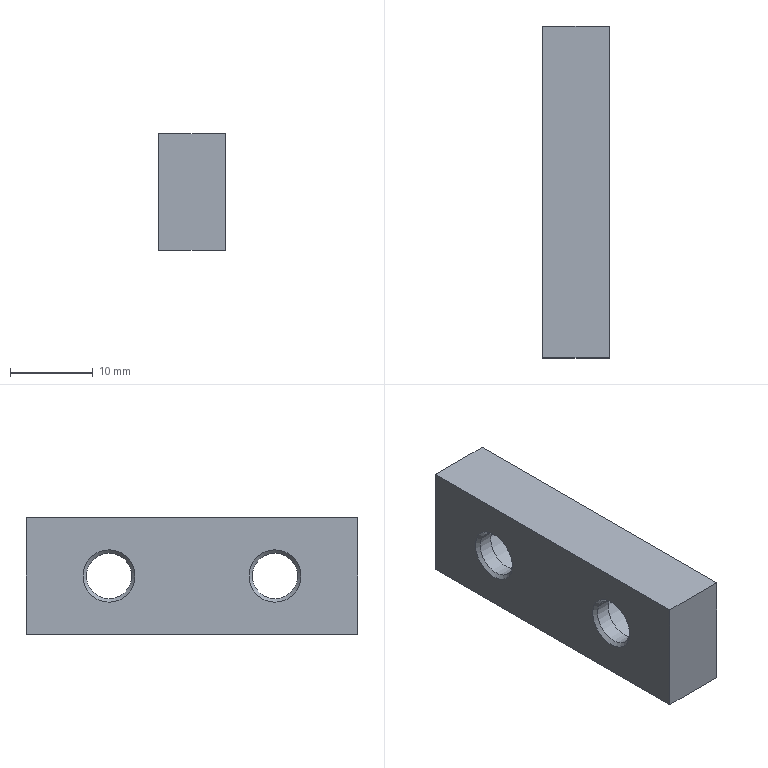Component | NX | A_SUPPORT_PLATE_2 | 1 solid | 16 faces | box 8 x 40 x 14 mm | volume 3456 mm3 | plane 8 | cylinder 4 | cone 4 | commonest cylinder face diameters 5.5 x2 10 x2
STEP:
#1=CARTESIAN_POINT('',(0.,0.,0.));
#2=DIRECTION('',(0.,0.,1.));
#3=DIRECTION('',(1.,0.,0.));
#4=AXIS2_PLACEMENT_3D('',#1,#2,#3);
#5=CARTESIAN_POINT('',(-25.,-20.,12.5));
#6=VERTEX_POINT('',#5);
#7=CARTESIAN_POINT('',(-25.,-20.,-1.5));
#8=VERTEX_POINT('',#7);
#9=CARTESIAN_POINT('',(-25.,-20.,12.5));
#10=DIRECTION('',(0.,0.,-1.));
#11=VECTOR('',#10,1.);
#12=LINE('',#9,#11);
#13=CARTESIAN_POINT('',(-33.,-20.,12.5));
#14=DIRECTION('',(0.,-1.,0.));
#15=DIRECTION('',(0.,0.,-1.));
#16=AXIS2_PLACEMENT_3D('',#13,#14,#15);
#17=PLANE('',#16);
#18=CARTESIAN_POINT('',(0.,8.));
#19=DIRECTION('',(1.,0.));
#20=VECTOR('',#19,1.);
#21=LINE('',#18,#20);
#22=(GEOMETRIC_REPRESENTATION_CONTEXT(2)PARAMETRIC_REPRESENTATION_CONTEXT()REPRESENTATION_CONTEXT('',''));
#23=DEFINITIONAL_REPRESENTATION('',(#21),#22);
#24=PCURVE('',#17,#23);
#25=CARTESIAN_POINT('',(-25.,0.,5.5));
#26=DIRECTION('',(1.,0.,0.));
#27=DIRECTION('',(0.,0.,-1.));
#28=AXIS2_PLACEMENT_3D('',#25,#26,#27);
#29=PLANE('',#28);
#30=CARTESIAN_POINT('',(-7.,-20.));
#31=DIRECTION('',(1.,0.));
#32=VECTOR('',#31,1.);
#33=LINE('',#30,#32);
#34=(GEOMETRIC_REPRESENTATION_CONTEXT(2)PARAMETRIC_REPRESENTATION_CONTEXT()REPRESENTATION_CONTEXT('',''));
#35=DEFINITIONAL_REPRESENTATION('',(#33),#34);
#36=PCURVE('',#29,#35);
#37=SURFACE_CURVE('',#12,(#24,#36),.PCURVE_S1.);
#38=EDGE_CURVE('',#6,#8,#37,.T.);
#39=ORIENTED_EDGE('',*,*,#38,.F.);
#40=CARTESIAN_POINT('',(-33.,-20.,12.5));
#41=VERTEX_POINT('',#40);
#42=CARTESIAN_POINT('',(-33.,-20.,12.5));
#43=DIRECTION('',(1.,0.,0.));
#44=VECTOR('',#43,1.);
#45=LINE('',#42,#44);
#46=CARTESIAN_POINT('',(0.,0.));
#47=DIRECTION('',(0.,1.));
#48=VECTOR('',#47,1.);
#49=LINE('',#46,#48);
#50=(GEOMETRIC_REPRESENTATION_CONTEXT(2)PARAMETRIC_REPRESENTATION_CONTEXT()REPRESENTATION_CONTEXT('',''));
#51=DEFINITIONAL_REPRESENTATION('',(#49),#50);
#52=PCURVE('',#17,#51);
#53=CARTESIAN_POINT('',(-33.,20.,12.5));
#54=DIRECTION('',(0.,0.,1.));
#55=DIRECTION('',(1.,0.,0.));
#56=AXIS2_PLACEMENT_3D('',#53,#54,#55);
#57=PLANE('',#56);
#58=CARTESIAN_POINT('',(0.,-40.));
#59=DIRECTION('',(1.,0.));
#60=VECTOR('',#59,1.);
#61=LINE('',#58,#60);
#62=(GEOMETRIC_REPRESENTATION_CONTEXT(2)PARAMETRIC_REPRESENTATION_CONTEXT()REPRESENTATION_CONTEXT('',''));
#63=DEFINITIONAL_REPRESENTATION('',(#61),#62);
#64=PCURVE('',#57,#63);
#65=SURFACE_CURVE('',#45,(#52,#64),.PCURVE_S1.);
#66=EDGE_CURVE('',#41,#6,#65,.T.);
#67=ORIENTED_EDGE('',*,*,#66,.F.);
#68=CARTESIAN_POINT('',(-33.,-20.,-1.5));
#69=VERTEX_POINT('',#68);
#70=CARTESIAN_POINT('',(-33.,-20.,12.5));
#71=DIRECTION('',(0.,0.,-1.));
#72=VECTOR('',#71,1.);
#73=LINE('',#70,#72);
#74=CARTESIAN_POINT('',(0.,0.));
#75=DIRECTION('',(1.,0.));
#76=VECTOR('',#75,1.);
#77=LINE('',#74,#76);
#78=(GEOMETRIC_REPRESENTATION_CONTEXT(2)PARAMETRIC_REPRESENTATION_CONTEXT()REPRESENTATION_CONTEXT('',''));
#79=DEFINITIONAL_REPRESENTATION('',(#77),#78);
#80=PCURVE('',#17,#79);
#81=CARTESIAN_POINT('',(-33.,0.,5.5));
#82=DIRECTION('',(1.,0.,0.));
#83=DIRECTION('',(0.,0.,-1.));
#84=AXIS2_PLACEMENT_3D('',#81,#82,#83);
#85=PLANE('',#84);
#86=CARTESIAN_POINT('',(-7.,-20.));
#87=DIRECTION('',(1.,0.));
#88=VECTOR('',#87,1.);
#89=LINE('',#86,#88);
#90=(GEOMETRIC_REPRESENTATION_CONTEXT(2)PARAMETRIC_REPRESENTATION_CONTEXT()REPRESENTATION_CONTEXT('',''));
#91=DEFINITIONAL_REPRESENTATION('',(#89),#90);
#92=PCURVE('',#85,#91);
#93=SURFACE_CURVE('',#73,(#80,#92),.PCURVE_S1.);
#94=EDGE_CURVE('',#41,#69,#93,.T.);
#95=ORIENTED_EDGE('',*,*,#94,.T.);
#96=CARTESIAN_POINT('',(-33.,-20.,-1.5));
#97=DIRECTION('',(1.,0.,0.));
#98=VECTOR('',#97,1.);
#99=LINE('',#96,#98);
#100=CARTESIAN_POINT('',(14.,0.));
#101=DIRECTION('',(0.,1.));
#102=VECTOR('',#101,1.);
#103=LINE('',#100,#102);
#104=(GEOMETRIC_REPRESENTATION_CONTEXT(2)PARAMETRIC_REPRESENTATION_CONTEXT()REPRESENTATION_CONTEXT('',''));
#105=DEFINITIONAL_REPRESENTATION('',(#103),#104);
#106=PCURVE('',#17,#105);
#107=CARTESIAN_POINT('',(-33.,-20.,-1.5));
#108=DIRECTION('',(0.,0.,-1.));
#109=DIRECTION('',(-1.,0.,0.));
#110=AXIS2_PLACEMENT_3D('',#107,#108,#109);
#111=PLANE('',#110);
#112=CARTESIAN_POINT('',(0.,0.));
#113=DIRECTION('',(-1.,0.));
#114=VECTOR('',#113,1.);
#115=LINE('',#112,#114);
#116=(GEOMETRIC_REPRESENTATION_CONTEXT(2)PARAMETRIC_REPRESENTATION_CONTEXT()REPRESENTATION_CONTEXT('',''));
#117=DEFINITIONAL_REPRESENTATION('',(#115),#116);
#118=PCURVE('',#111,#117);
#119=SURFACE_CURVE('',#99,(#106,#118),.PCURVE_S1.);
#120=EDGE_CURVE('',#69,#8,#119,.T.);
#121=ORIENTED_EDGE('',*,*,#120,.T.);
#122=EDGE_LOOP('',(#39,#67,#95,#121));
#123=FACE_BOUND('',#122,.T.);
#124=ADVANCED_FACE('',(#123),#17,.T.);
#125=CARTESIAN_POINT('',(-25.,20.,-1.5));
#126=VERTEX_POINT('',#125);
#127=CARTESIAN_POINT('',(-25.,-20.,-1.5));
#128=DIRECTION('',(0.,1.,0.));
#129=VECTOR('',#128,1.);
#130=LINE('',#127,#129);
#131=CARTESIAN_POINT('',(-8.,0.));
#132=DIRECTION('',(0.,1.));
#133=VECTOR('',#132,1.);
#134=LINE('',#131,#133);
#135=(GEOMETRIC_REPRESENTATION_CONTEXT(2)PARAMETRIC_REPRESENTATION_CONTEXT()REPRESENTATION_CONTEXT('',''));
#136=DEFINITIONAL_REPRESENTATION('',(#134),#135);
#137=PCURVE('',#111,#136);
#138=CARTESIAN_POINT('',(7.,-20.));
#139=DIRECTION('',(0.,1.));
#140=VECTOR('',#139,1.);
#141=LINE('',#138,#140);
#142=(GEOMETRIC_REPRESENTATION_CONTEXT(2)PARAMETRIC_REPRESENTATION_CONTEXT()REPRESENTATION_CONTEXT('',''));
#143=DEFINITIONAL_REPRESENTATION('',(#141),#142);
#144=PCURVE('',#29,#143);
#145=SURFACE_CURVE('',#130,(#137,#144),.PCURVE_S1.);
#146=EDGE_CURVE('',#8,#126,#145,.T.);
#147=ORIENTED_EDGE('',*,*,#146,.F.);
#148=ORIENTED_EDGE('',*,*,#120,.F.);
#149=CARTESIAN_POINT('',(-33.,20.,-1.5));
#150=VERTEX_POINT('',#149);
#151=CARTESIAN_POINT('',(-33.,-20.,-1.5));
#152=DIRECTION('',(0.,1.,0.));
#153=VECTOR('',#152,1.);
#154=LINE('',#151,#153);
#155=CARTESIAN_POINT('',(0.,0.));
#156=DIRECTION('',(0.,1.));
#157=VECTOR('',#156,1.);
#158=LINE('',#155,#157);
#159=(GEOMETRIC_REPRESENTATION_CONTEXT(2)PARAMETRIC_REPRESENTATION_CONTEXT()REPRESENTATION_CONTEXT('',''));
#160=DEFINITIONAL_REPRESENTATION('',(#158),#159);
#161=PCURVE('',#111,#160);
#162=CARTESIAN_POINT('',(7.,-20.));
#163=DIRECTION('',(0.,1.));
#164=VECTOR('',#163,1.);
#165=LINE('',#162,#164);
#166=(GEOMETRIC_REPRESENTATION_CONTEXT(2)PARAMETRIC_REPRESENTATION_CONTEXT()REPRESENTATION_CONTEXT('',''));
#167=DEFINITIONAL_REPRESENTATION('',(#165),#166);
#168=PCURVE('',#85,#167);
#169=SURFACE_CURVE('',#154,(#161,#168),.PCURVE_S1.);
#170=EDGE_CURVE('',#69,#150,#169,.T.);
#171=ORIENTED_EDGE('',*,*,#170,.T.);
#172=CARTESIAN_POINT('',(-33.,20.,-1.5));
#173=DIRECTION('',(1.,0.,0.));
#174=VECTOR('',#173,1.);
#175=LINE('',#172,#174);
#176=CARTESIAN_POINT('',(0.,40.));
#177=DIRECTION('',(-1.,0.));
#178=VECTOR('',#177,1.);
#179=LINE('',#176,#178);
#180=(GEOMETRIC_REPRESENTATION_CONTEXT(2)PARAMETRIC_REPRESENTATION_CONTEXT()REPRESENTATION_CONTEXT('',''));
#181=DEFINITIONAL_REPRESENTATION('',(#179),#180);
#182=PCURVE('',#111,#181);
#183=CARTESIAN_POINT('',(-33.,20.,-1.5));
#184=DIRECTION('',(0.,1.,0.));
#185=DIRECTION('',(0.,0.,1.));
#186=AXIS2_PLACEMENT_3D('',#183,#184,#185);
#187=PLANE('',#186);
#188=CARTESIAN_POINT('',(0.,0.));
#189=DIRECTION('',(0.,1.));
#190=VECTOR('',#189,1.);
#191=LINE('',#188,#190);
#192=(GEOMETRIC_REPRESENTATION_CONTEXT(2)PARAMETRIC_REPRESENTATION_CONTEXT()REPRESENTATION_CONTEXT('',''));
#193=DEFINITIONAL_REPRESENTATION('',(#191),#192);
#194=PCURVE('',#187,#193);
#195=SURFACE_CURVE('',#175,(#182,#194),.PCURVE_S1.);
#196=EDGE_CURVE('',#150,#126,#195,.T.);
#197=ORIENTED_EDGE('',*,*,#196,.T.);
#198=EDGE_LOOP('',(#147,#148,#171,#197));
#199=FACE_BOUND('',#198,.T.);
#200=ADVANCED_FACE('',(#199),#111,.T.);
#201=CARTESIAN_POINT('',(-25.,20.,12.5));
#202=VERTEX_POINT('',#201);
#203=CARTESIAN_POINT('',(-25.,20.,-1.5));
#204=DIRECTION('',(0.,0.,1.));
#205=VECTOR('',#204,1.);
#206=LINE('',#203,#205);
#207=CARTESIAN_POINT('',(0.,8.));
#208=DIRECTION('',(1.,0.));
#209=VECTOR('',#208,1.);
#210=LINE('',#207,#209);
#211=(GEOMETRIC_REPRESENTATION_CONTEXT(2)PARAMETRIC_REPRESENTATION_CONTEXT()REPRESENTATION_CONTEXT('',''));
#212=DEFINITIONAL_REPRESENTATION('',(#210),#211);
#213=PCURVE('',#187,#212);
#214=CARTESIAN_POINT('',(7.,20.));
#215=DIRECTION('',(-1.,0.));
#216=VECTOR('',#215,1.);
#217=LINE('',#214,#216);
#218=(GEOMETRIC_REPRESENTATION_CONTEXT(2)PARAMETRIC_REPRESENTATION_CONTEXT()REPRESENTATION_CONTEXT('',''));
#219=DEFINITIONAL_REPRESENTATION('',(#217),#218);
#220=PCURVE('',#29,#219);
#221=SURFACE_CURVE('',#206,(#213,#220),.PCURVE_S1.);
#222=EDGE_CURVE('',#126,#202,#221,.T.);
#223=ORIENTED_EDGE('',*,*,#222,.F.);
#224=ORIENTED_EDGE('',*,*,#196,.F.);
#225=CARTESIAN_POINT('',(-33.,20.,12.5));
#226=VERTEX_POINT('',#225);
#227=CARTESIAN_POINT('',(-33.,20.,-1.5));
#228=DIRECTION('',(0.,0.,1.));
#229=VECTOR('',#228,1.);
#230=LINE('',#227,#229);
#231=CARTESIAN_POINT('',(0.,0.));
#232=DIRECTION('',(1.,0.));
#233=VECTOR('',#232,1.);
#234=LINE('',#231,#233);
#235=(GEOMETRIC_REPRESENTATION_CONTEXT(2)PARAMETRIC_REPRESENTATION_CONTEXT()REPRESENTATION_CONTEXT('',''));
#236=DEFINITIONAL_REPRESENTATION('',(#234),#235);
#237=PCURVE('',#187,#236);
#238=CARTESIAN_POINT('',(7.,20.));
#239=DIRECTION('',(-1.,0.));
#240=VECTOR('',#239,1.);
#241=LINE('',#238,#240);
#242=(GEOMETRIC_REPRESENTATION_CONTEXT(2)PARAMETRIC_REPRESENTATION_CONTEXT()REPRESENTATION_CONTEXT('',''));
#243=DEFINITIONAL_REPRESENTATION('',(#241),#242);
#244=PCURVE('',#85,#243);
#245=SURFACE_CURVE('',#230,(#237,#244),.PCURVE_S1.);
#246=EDGE_CURVE('',#150,#226,#245,.T.);
#247=ORIENTED_EDGE('',*,*,#246,.T.);
#248=CARTESIAN_POINT('',(-33.,20.,12.5));
#249=DIRECTION('',(1.,0.,0.));
#250=VECTOR('',#249,1.);
#251=LINE('',#248,#250);
#252=CARTESIAN_POINT('',(14.,0.));
#253=DIRECTION('',(0.,1.));
#254=VECTOR('',#253,1.);
#255=LINE('',#252,#254);
#256=(GEOMETRIC_REPRESENTATION_CONTEXT(2)PARAMETRIC_REPRESENTATION_CONTEXT()REPRESENTATION_CONTEXT('',''));
#257=DEFINITIONAL_REPRESENTATION('',(#255),#256);
#258=PCURVE('',#187,#257);
#259=CARTESIAN_POINT('',(0.,0.));
#260=DIRECTION('',(1.,0.));
#261=VECTOR('',#260,1.);
#262=LINE('',#259,#261);
#263=(GEOMETRIC_REPRESENTATION_CONTEXT(2)PARAMETRIC_REPRESENTATION_CONTEXT()REPRESENTATION_CONTEXT('',''));
#264=DEFINITIONAL_REPRESENTATION('',(#262),#263);
#265=PCURVE('',#57,#264);
#266=SURFACE_CURVE('',#251,(#258,#265),.PCURVE_S1.);
#267=EDGE_CURVE('',#226,#202,#266,.T.);
#268=ORIENTED_EDGE('',*,*,#267,.T.);
#269=EDGE_LOOP('',(#223,#224,#247,#268));
#270=FACE_BOUND('',#269,.T.);
#271=ADVANCED_FACE('',(#270),#187,.T.);
#272=CARTESIAN_POINT('',(-25.,20.,12.5));
#273=DIRECTION('',(0.,-1.,0.));
#274=VECTOR('',#273,1.);
#275=LINE('',#272,#274);
#276=CARTESIAN_POINT('',(8.,0.));
#277=DIRECTION('',(0.,-1.));
#278=VECTOR('',#277,1.);
#279=LINE('',#276,#278);
#280=(GEOMETRIC_REPRESENTATION_CONTEXT(2)PARAMETRIC_REPRESENTATION_CONTEXT()REPRESENTATION_CONTEXT('',''));
#281=DEFINITIONAL_REPRESENTATION('',(#279),#280);
#282=PCURVE('',#57,#281);
#283=CARTESIAN_POINT('',(-7.,20.));
#284=DIRECTION('',(0.,-1.));
#285=VECTOR('',#284,1.);
#286=LINE('',#283,#285);
#287=(GEOMETRIC_REPRESENTATION_CONTEXT(2)PARAMETRIC_REPRESENTATION_CONTEXT()REPRESENTATION_CONTEXT('',''));
#288=DEFINITIONAL_REPRESENTATION('',(#286),#287);
#289=PCURVE('',#29,#288);
#290=SURFACE_CURVE('',#275,(#282,#289),.PCURVE_S1.);
#291=EDGE_CURVE('',#202,#6,#290,.T.);
#292=ORIENTED_EDGE('',*,*,#291,.F.);
#293=ORIENTED_EDGE('',*,*,#267,.F.);
#294=CARTESIAN_POINT('',(-33.,20.,12.5));
#295=DIRECTION('',(0.,-1.,0.));
#296=VECTOR('',#295,1.);
#297=LINE('',#294,#296);
#298=CARTESIAN_POINT('',(0.,0.));
#299=DIRECTION('',(0.,-1.));
#300=VECTOR('',#299,1.);
#301=LINE('',#298,#300);
#302=(GEOMETRIC_REPRESENTATION_CONTEXT(2)PARAMETRIC_REPRESENTATION_CONTEXT()REPRESENTATION_CONTEXT('',''));
#303=DEFINITIONAL_REPRESENTATION('',(#301),#302);
#304=PCURVE('',#57,#303);
#305=CARTESIAN_POINT('',(-7.,20.));
#306=DIRECTION('',(0.,-1.));
#307=VECTOR('',#306,1.);
#308=LINE('',#305,#307);
#309=(GEOMETRIC_REPRESENTATION_CONTEXT(2)PARAMETRIC_REPRESENTATION_CONTEXT()REPRESENTATION_CONTEXT('',''));
#310=DEFINITIONAL_REPRESENTATION('',(#308),#309);
#311=PCURVE('',#85,#310);
#312=SURFACE_CURVE('',#297,(#304,#311),.PCURVE_S1.);
#313=EDGE_CURVE('',#226,#41,#312,.T.);
#314=ORIENTED_EDGE('',*,*,#313,.T.);
#315=ORIENTED_EDGE('',*,*,#66,.T.);
#316=EDGE_LOOP('',(#292,#293,#314,#315));
#317=FACE_BOUND('',#316,.T.);
#318=ADVANCED_FACE('',(#317),#57,.T.);
#319=CARTESIAN_POINT('',(-33.,10.,2.35));
#320=VERTEX_POINT('',#319);
#321=CARTESIAN_POINT('',(-33.,10.,5.5));
#322=DIRECTION('',(1.,0.,0.));
#323=DIRECTION('',(0.,0.,-1.));
#324=AXIS2_PLACEMENT_3D('',#321,#322,#323);
#325=CIRCLE('',#324,3.15);
#326=CARTESIAN_POINT('',(0.,10.));
#327=DIRECTION('',(1.,0.));
#328=AXIS2_PLACEMENT_2D('',#326,#327);
#329=CIRCLE('',#328,3.15);
#330=(GEOMETRIC_REPRESENTATION_CONTEXT(2)PARAMETRIC_REPRESENTATION_CONTEXT()REPRESENTATION_CONTEXT('',''));
#331=DEFINITIONAL_REPRESENTATION('',(#329),#330);
#332=PCURVE('',#85,#331);
#333=CARTESIAN_POINT('',(-33.,10.,5.5));
#334=DIRECTION('',(-1.,0.,0.));
#335=DIRECTION('',(0.,0.,1.));
#336=AXIS2_PLACEMENT_3D('',#333,#334,#335);
#337=CONICAL_SURFACE('',#336,3.15,0.7854);
#338=CARTESIAN_POINT('',(9.425,0.));
#339=DIRECTION('',(-1.,0.));
#340=VECTOR('',#339,1.);
#341=LINE('',#338,#340);
#342=(GEOMETRIC_REPRESENTATION_CONTEXT(2)PARAMETRIC_REPRESENTATION_CONTEXT()REPRESENTATION_CONTEXT('',''));
#343=DEFINITIONAL_REPRESENTATION('',(#341),#342);
#344=PCURVE('',#337,#343);
#345=SURFACE_CURVE('',#325,(#332,#344),.PCURVE_S1.);
#346=EDGE_CURVE('',#320,#320,#345,.T.);
#347=ORIENTED_EDGE('',*,*,#346,.T.);
#348=EDGE_LOOP('',(#347));
#349=FACE_BOUND('',#348,.T.);
#350=CARTESIAN_POINT('',(-33.,-10.,2.35));
#351=VERTEX_POINT('',#350);
#352=CARTESIAN_POINT('',(-33.,-10.,5.5));
#353=DIRECTION('',(1.,0.,0.));
#354=DIRECTION('',(0.,0.,-1.));
#355=AXIS2_PLACEMENT_3D('',#352,#353,#354);
#356=CIRCLE('',#355,3.15);
#357=CARTESIAN_POINT('',(0.,-10.));
#358=DIRECTION('',(1.,0.));
#359=AXIS2_PLACEMENT_2D('',#357,#358);
#360=CIRCLE('',#359,3.15);
#361=(GEOMETRIC_REPRESENTATION_CONTEXT(2)PARAMETRIC_REPRESENTATION_CONTEXT()REPRESENTATION_CONTEXT('',''));
#362=DEFINITIONAL_REPRESENTATION('',(#360),#361);
#363=PCURVE('',#85,#362);
#364=CARTESIAN_POINT('',(-33.,-10.,5.5));
#365=DIRECTION('',(-1.,0.,0.));
#366=DIRECTION('',(0.,0.,1.));
#367=AXIS2_PLACEMENT_3D('',#364,#365,#366);
#368=CONICAL_SURFACE('',#367,3.15,0.7854);
#369=CARTESIAN_POINT('',(9.425,0.));
#370=DIRECTION('',(-1.,0.));
#371=VECTOR('',#370,1.);
#372=LINE('',#369,#371);
#373=(GEOMETRIC_REPRESENTATION_CONTEXT(2)PARAMETRIC_REPRESENTATION_CONTEXT()REPRESENTATION_CONTEXT('',''));
#374=DEFINITIONAL_REPRESENTATION('',(#372),#373);
#375=PCURVE('',#368,#374);
#376=SURFACE_CURVE('',#356,(#363,#375),.PCURVE_S1.);
#377=EDGE_CURVE('',#351,#351,#376,.T.);
#378=ORIENTED_EDGE('',*,*,#377,.T.);
#379=EDGE_LOOP('',(#378));
#380=FACE_BOUND('',#379,.T.);
#381=ORIENTED_EDGE('',*,*,#94,.F.);
#382=ORIENTED_EDGE('',*,*,#313,.F.);
#383=ORIENTED_EDGE('',*,*,#246,.F.);
#384=ORIENTED_EDGE('',*,*,#170,.F.);
#385=EDGE_LOOP('',(#381,#382,#383,#384));
#386=FACE_BOUND('',#385,.T.);
#387=ADVANCED_FACE('',(#349,#380,#386),#85,.F.);
#388=CARTESIAN_POINT('',(-25.,10.,0.1));
#389=VERTEX_POINT('',#388);
#390=CARTESIAN_POINT('',(-25.,10.,5.5));
#391=DIRECTION('',(-1.,0.,0.));
#392=DIRECTION('',(0.,0.,-1.));
#393=AXIS2_PLACEMENT_3D('',#390,#391,#392);
#394=CIRCLE('',#393,5.4);
#395=CARTESIAN_POINT('',(5.4,10.));
#396=CARTESIAN_POINT('',(5.4,0.6469));
#397=CARTESIAN_POINT('',(-2.7,5.323));
#398=CARTESIAN_POINT('',(-10.8,10.));
#399=CARTESIAN_POINT('',(-2.7,14.677));
#400=CARTESIAN_POINT('',(5.4,19.353));
#401=CARTESIAN_POINT('',(5.4,10.));
#402=(BOUNDED_CURVE()B_SPLINE_CURVE(2,(#395,#396,#397,#398,#399,#400,#401),.UNSPECIFIED.,.T.,.F.)B_SPLINE_CURVE_WITH_KNOTS((1,2,2,2,2,1),(-2.094,0.,2.094,4.189,6.283,8.378),.UNSPECIFIED.)CURVE()GEOMETRIC_REPRESENTATION_ITEM()RATIONAL_B_SPLINE_CURVE((1.,0.5,1.,0.5,1.,0.5,1.))REPRESENTATION_ITEM(''));
#403=(GEOMETRIC_REPRESENTATION_CONTEXT(2)PARAMETRIC_REPRESENTATION_CONTEXT()REPRESENTATION_CONTEXT('',''));
#404=DEFINITIONAL_REPRESENTATION('',(#402),#403);
#405=PCURVE('',#29,#404);
#406=CARTESIAN_POINT('',(-25.,10.,5.5));
#407=DIRECTION('',(1.,0.,0.));
#408=DIRECTION('',(0.,0.,-1.));
#409=AXIS2_PLACEMENT_3D('',#406,#407,#408);
#410=CONICAL_SURFACE('',#409,5.4,0.7854);
#411=CARTESIAN_POINT('',(6.283,0.));
#412=DIRECTION('',(-1.,0.));
#413=VECTOR('',#412,1.);
#414=LINE('',#411,#413);
#415=(GEOMETRIC_REPRESENTATION_CONTEXT(2)PARAMETRIC_REPRESENTATION_CONTEXT()REPRESENTATION_CONTEXT('',''));
#416=DEFINITIONAL_REPRESENTATION('',(#414),#415);
#417=PCURVE('',#410,#416);
#418=SURFACE_CURVE('',#394,(#405,#417),.PCURVE_S1.);
#419=EDGE_CURVE('',#389,#389,#418,.T.);
#420=ORIENTED_EDGE('',*,*,#419,.T.);
#421=EDGE_LOOP('',(#420));
#422=FACE_BOUND('',#421,.T.);
#423=CARTESIAN_POINT('',(-25.,-10.,0.1));
#424=VERTEX_POINT('',#423);
#425=CARTESIAN_POINT('',(-25.,-10.,5.5));
#426=DIRECTION('',(-1.,0.,0.));
#427=DIRECTION('',(0.,0.,-1.));
#428=AXIS2_PLACEMENT_3D('',#425,#426,#427);
#429=CIRCLE('',#428,5.4);
#430=CARTESIAN_POINT('',(5.4,-10.));
#431=CARTESIAN_POINT('',(5.4,-19.353));
#432=CARTESIAN_POINT('',(-2.7,-14.677));
#433=CARTESIAN_POINT('',(-10.8,-10.));
#434=CARTESIAN_POINT('',(-2.7,-5.323));
#435=CARTESIAN_POINT('',(5.4,-0.6469));
#436=CARTESIAN_POINT('',(5.4,-10.));
#437=(BOUNDED_CURVE()B_SPLINE_CURVE(2,(#430,#431,#432,#433,#434,#435,#436),.UNSPECIFIED.,.T.,.F.)B_SPLINE_CURVE_WITH_KNOTS((1,2,2,2,2,1),(-2.094,0.,2.094,4.189,6.283,8.378),.UNSPECIFIED.)CURVE()GEOMETRIC_REPRESENTATION_ITEM()RATIONAL_B_SPLINE_CURVE((1.,0.5,1.,0.5,1.,0.5,1.))REPRESENTATION_ITEM(''));
#438=(GEOMETRIC_REPRESENTATION_CONTEXT(2)PARAMETRIC_REPRESENTATION_CONTEXT()REPRESENTATION_CONTEXT('',''));
#439=DEFINITIONAL_REPRESENTATION('',(#437),#438);
#440=PCURVE('',#29,#439);
#441=CARTESIAN_POINT('',(-25.,-10.,5.5));
#442=DIRECTION('',(1.,0.,0.));
#443=DIRECTION('',(0.,0.,-1.));
#444=AXIS2_PLACEMENT_3D('',#441,#442,#443);
#445=CONICAL_SURFACE('',#444,5.4,0.7854);
#446=CARTESIAN_POINT('',(6.283,0.));
#447=DIRECTION('',(-1.,0.));
#448=VECTOR('',#447,1.);
#449=LINE('',#446,#448);
#450=(GEOMETRIC_REPRESENTATION_CONTEXT(2)PARAMETRIC_REPRESENTATION_CONTEXT()REPRESENTATION_CONTEXT('',''));
#451=DEFINITIONAL_REPRESENTATION('',(#449),#450);
#452=PCURVE('',#445,#451);
#453=SURFACE_CURVE('',#429,(#440,#452),.PCURVE_S1.);
#454=EDGE_CURVE('',#424,#424,#453,.T.);
#455=ORIENTED_EDGE('',*,*,#454,.T.);
#456=EDGE_LOOP('',(#455));
#457=FACE_BOUND('',#456,.T.);
#458=ORIENTED_EDGE('',*,*,#38,.T.);
#459=ORIENTED_EDGE('',*,*,#146,.T.);
#460=ORIENTED_EDGE('',*,*,#222,.T.);
#461=ORIENTED_EDGE('',*,*,#291,.T.);
#462=EDGE_LOOP('',(#458,#459,#460,#461));
#463=FACE_BOUND('',#462,.T.);
#464=ADVANCED_FACE('',(#422,#457,#463),#29,.T.);
#465=CARTESIAN_POINT('',(-32.6,-10.,8.25));
#466=VERTEX_POINT('',#465);
#467=CARTESIAN_POINT('',(-32.6,-10.,2.75));
#468=VERTEX_POINT('',#467);
#469=CARTESIAN_POINT('',(-32.6,-10.,5.5));
#470=DIRECTION('',(-1.,0.,0.));
#471=DIRECTION('',(0.,0.,-1.));
#472=AXIS2_PLACEMENT_3D('',#469,#470,#471);
#473=CIRCLE('',#472,2.75);
#474=CARTESIAN_POINT('',(-50.509,-10.,5.5));
#475=DIRECTION('',(-1.,0.,0.));
#476=DIRECTION('',(0.,0.,1.));
#477=AXIS2_PLACEMENT_3D('',#474,#475,#476);
#478=CYLINDRICAL_SURFACE('',#477,2.75);
#479=CARTESIAN_POINT('',(-3.142,-17.909));
#480=DIRECTION('',(1.,0.));
#481=VECTOR('',#480,1.);
#482=LINE('',#479,#481);
#483=(GEOMETRIC_REPRESENTATION_CONTEXT(2)PARAMETRIC_REPRESENTATION_CONTEXT()REPRESENTATION_CONTEXT('',''));
#484=DEFINITIONAL_REPRESENTATION('',(#482),#483);
#485=PCURVE('',#478,#484);
#486=CARTESIAN_POINT('',(3.142,-0.4));
#487=DIRECTION('',(1.,0.));
#488=VECTOR('',#487,1.);
#489=LINE('',#486,#488);
#490=(GEOMETRIC_REPRESENTATION_CONTEXT(2)PARAMETRIC_REPRESENTATION_CONTEXT()REPRESENTATION_CONTEXT('',''));
#491=DEFINITIONAL_REPRESENTATION('',(#489),#490);
#492=PCURVE('',#368,#491);
#493=SURFACE_CURVE('',#473,(#485,#492),.PCURVE_S1.);
#494=EDGE_CURVE('',#466,#468,#493,.T.);
#495=ORIENTED_EDGE('',*,*,#494,.F.);
#496=CARTESIAN_POINT('',(-30.8,-10.,8.25));
#497=VERTEX_POINT('',#496);
#498=CARTESIAN_POINT('',(-30.8,-10.,8.25));
#499=CARTESIAN_POINT('',(-32.6,-10.,8.25));
#500=B_SPLINE_CURVE_WITH_KNOTS('',1,(#498,#499),.UNSPECIFIED.,.F.,.F.,(2,2),(-19.709,-17.909),.PIECEWISE_BEZIER_KNOTS.);
#501=CARTESIAN_POINT('',(0.,0.));
#502=DIRECTION('',(0.,1.));
#503=VECTOR('',#502,1.);
#504=LINE('',#501,#503);
#505=(GEOMETRIC_REPRESENTATION_CONTEXT(2)PARAMETRIC_REPRESENTATION_CONTEXT()REPRESENTATION_CONTEXT('',''));
#506=DEFINITIONAL_REPRESENTATION('',(#504),#505);
#507=PCURVE('',#478,#506);
#508=CARTESIAN_POINT('',(6.283,0.));
#509=DIRECTION('',(0.,1.));
#510=VECTOR('',#509,1.);
#511=LINE('',#508,#510);
#512=(GEOMETRIC_REPRESENTATION_CONTEXT(2)PARAMETRIC_REPRESENTATION_CONTEXT()REPRESENTATION_CONTEXT('',''));
#513=DEFINITIONAL_REPRESENTATION('',(#511),#512);
#514=PCURVE('',#478,#513);
#515=SEAM_CURVE('',#500,(#507,#514),.PCURVE_S1.);
#516=EDGE_CURVE('',#497,#466,#515,.T.);
#517=ORIENTED_EDGE('',*,*,#516,.F.);
#518=CARTESIAN_POINT('',(-30.8,-10.,5.5));
#519=DIRECTION('',(1.,0.,0.));
#520=DIRECTION('',(0.,0.,1.));
#521=AXIS2_PLACEMENT_3D('',#518,#519,#520);
#522=CIRCLE('',#521,2.75);
#523=CARTESIAN_POINT('',(6.283,-19.709));
#524=DIRECTION('',(-1.,0.));
#525=VECTOR('',#524,1.);
#526=LINE('',#523,#525);
#527=(GEOMETRIC_REPRESENTATION_CONTEXT(2)PARAMETRIC_REPRESENTATION_CONTEXT()REPRESENTATION_CONTEXT('',''));
#528=DEFINITIONAL_REPRESENTATION('',(#526),#527);
#529=PCURVE('',#478,#528);
#530=CARTESIAN_POINT('',(-30.8,-10.,5.5));
#531=DIRECTION('',(-1.,0.,0.));
#532=DIRECTION('',(0.,0.,1.));
#533=AXIS2_PLACEMENT_3D('',#530,#531,#532);
#534=PLANE('',#533);
#535=CARTESIAN_POINT('',(2.75,0.));
#536=CARTESIAN_POINT('',(2.75,-4.763));
#537=CARTESIAN_POINT('',(-1.375,-2.382));
#538=CARTESIAN_POINT('',(-5.5,-0.));
#539=CARTESIAN_POINT('',(-1.375,2.382));
#540=CARTESIAN_POINT('',(2.75,4.763));
#541=CARTESIAN_POINT('',(2.75,0.));
#542=(BOUNDED_CURVE()B_SPLINE_CURVE(2,(#535,#536,#537,#538,#539,#540,#541),.UNSPECIFIED.,.T.,.F.)B_SPLINE_CURVE_WITH_KNOTS((1,2,2,2,2,1),(-2.094,0.,2.094,4.189,6.283,8.378),.UNSPECIFIED.)CURVE()GEOMETRIC_REPRESENTATION_ITEM()RATIONAL_B_SPLINE_CURVE((1.,0.5,1.,0.5,1.,0.5,1.))REPRESENTATION_ITEM(''));
#543=(GEOMETRIC_REPRESENTATION_CONTEXT(2)PARAMETRIC_REPRESENTATION_CONTEXT()REPRESENTATION_CONTEXT('',''));
#544=DEFINITIONAL_REPRESENTATION('',(#542),#543);
#545=PCURVE('',#534,#544);
#546=SURFACE_CURVE('',#522,(#529,#545),.PCURVE_S1.);
#547=EDGE_CURVE('',#497,#497,#546,.T.);
#548=ORIENTED_EDGE('',*,*,#547,.F.);
#549=ORIENTED_EDGE('',*,*,#516,.T.);
#550=CARTESIAN_POINT('',(-32.6,-10.,5.5));
#551=DIRECTION('',(-1.,0.,0.));
#552=DIRECTION('',(0.,0.,-1.));
#553=AXIS2_PLACEMENT_3D('',#550,#551,#552);
#554=CIRCLE('',#553,2.75);
#555=CARTESIAN_POINT('',(3.142,-17.909));
#556=DIRECTION('',(1.,0.));
#557=VECTOR('',#556,1.);
#558=LINE('',#555,#557);
#559=(GEOMETRIC_REPRESENTATION_CONTEXT(2)PARAMETRIC_REPRESENTATION_CONTEXT()REPRESENTATION_CONTEXT('',''));
#560=DEFINITIONAL_REPRESENTATION('',(#558),#559);
#561=PCURVE('',#478,#560);
#562=CARTESIAN_POINT('',(3.142,-0.4));
#563=DIRECTION('',(1.,-0.));
#564=VECTOR('',#563,1.);
#565=LINE('',#562,#564);
#566=(GEOMETRIC_REPRESENTATION_CONTEXT(2)PARAMETRIC_REPRESENTATION_CONTEXT()REPRESENTATION_CONTEXT('',''));
#567=DEFINITIONAL_REPRESENTATION('',(#565),#566);
#568=PCURVE('',#368,#567);
#569=SURFACE_CURVE('',#554,(#561,#568),.PCURVE_S1.);
#570=EDGE_CURVE('',#468,#466,#569,.T.);
#571=ORIENTED_EDGE('',*,*,#570,.F.);
#572=EDGE_LOOP('',(#495,#517,#548,#549,#571));
#573=FACE_BOUND('',#572,.F.);
#574=ADVANCED_FACE('',(#573),#478,.F.);
#575=ORIENTED_EDGE('',*,*,#547,.F.);
#576=EDGE_LOOP('',(#575));
#577=FACE_BOUND('',#576,.T.);
#578=CARTESIAN_POINT('',(-30.8,-10.,10.5));
#579=VERTEX_POINT('',#578);
#580=CARTESIAN_POINT('',(-30.8,-10.,5.5));
#581=DIRECTION('',(1.,0.,0.));
#582=DIRECTION('',(0.,0.,1.));
#583=AXIS2_PLACEMENT_3D('',#580,#581,#582);
#584=CIRCLE('',#583,5.);
#585=CARTESIAN_POINT('',(5.,0.));
#586=CARTESIAN_POINT('',(5.,-8.66));
#587=CARTESIAN_POINT('',(-2.5,-4.33));
#588=CARTESIAN_POINT('',(-10.,-0.));
#589=CARTESIAN_POINT('',(-2.5,4.33));
#590=CARTESIAN_POINT('',(5.,8.66));
#591=CARTESIAN_POINT('',(5.,0.));
#592=(BOUNDED_CURVE()B_SPLINE_CURVE(2,(#585,#586,#587,#588,#589,#590,#591),.UNSPECIFIED.,.T.,.F.)B_SPLINE_CURVE_WITH_KNOTS((1,2,2,2,2,1),(-2.094,0.,2.094,4.189,6.283,8.378),.UNSPECIFIED.)CURVE()GEOMETRIC_REPRESENTATION_ITEM()RATIONAL_B_SPLINE_CURVE((1.,0.5,1.,0.5,1.,0.5,1.))REPRESENTATION_ITEM(''));
#593=(GEOMETRIC_REPRESENTATION_CONTEXT(2)PARAMETRIC_REPRESENTATION_CONTEXT()REPRESENTATION_CONTEXT('',''));
#594=DEFINITIONAL_REPRESENTATION('',(#592),#593);
#595=PCURVE('',#534,#594);
#596=CARTESIAN_POINT('',(-25.,-10.,5.5));
#597=DIRECTION('',(-1.,0.,0.));
#598=DIRECTION('',(0.,0.,1.));
#599=AXIS2_PLACEMENT_3D('',#596,#597,#598);
#600=CYLINDRICAL_SURFACE('',#599,5.);
#601=CARTESIAN_POINT('',(6.283,5.8));
#602=DIRECTION('',(-1.,0.));
#603=VECTOR('',#602,1.);
#604=LINE('',#601,#603);
#605=(GEOMETRIC_REPRESENTATION_CONTEXT(2)PARAMETRIC_REPRESENTATION_CONTEXT()REPRESENTATION_CONTEXT('',''));
#606=DEFINITIONAL_REPRESENTATION('',(#604),#605);
#607=PCURVE('',#600,#606);
#608=SURFACE_CURVE('',#584,(#595,#607),.PCURVE_S1.);
#609=EDGE_CURVE('',#579,#579,#608,.T.);
#610=ORIENTED_EDGE('',*,*,#609,.T.);
#611=EDGE_LOOP('',(#610));
#612=FACE_BOUND('',#611,.T.);
#613=ADVANCED_FACE('',(#577,#612),#534,.F.);
#614=CARTESIAN_POINT('',(-25.4,-10.,10.5));
#615=VERTEX_POINT('',#614);
#616=CARTESIAN_POINT('',(-25.4,-10.,0.5));
#617=VERTEX_POINT('',#616);
#618=CARTESIAN_POINT('',(-25.4,-10.,5.5));
#619=DIRECTION('',(1.,0.,0.));
#620=DIRECTION('',(0.,0.,-1.));
#621=AXIS2_PLACEMENT_3D('',#618,#619,#620);
#622=CIRCLE('',#621,5.);
#623=CARTESIAN_POINT('',(9.425,0.4));
#624=DIRECTION('',(-1.,0.));
#625=VECTOR('',#624,1.);
#626=LINE('',#623,#625);
#627=(GEOMETRIC_REPRESENTATION_CONTEXT(2)PARAMETRIC_REPRESENTATION_CONTEXT()REPRESENTATION_CONTEXT('',''));
#628=DEFINITIONAL_REPRESENTATION('',(#626),#627);
#629=PCURVE('',#600,#628);
#630=CARTESIAN_POINT('',(0.,-0.4));
#631=DIRECTION('',(1.,0.));
#632=VECTOR('',#631,1.);
#633=LINE('',#630,#632);
#634=(GEOMETRIC_REPRESENTATION_CONTEXT(2)PARAMETRIC_REPRESENTATION_CONTEXT()REPRESENTATION_CONTEXT('',''));
#635=DEFINITIONAL_REPRESENTATION('',(#633),#634);
#636=PCURVE('',#445,#635);
#637=SURFACE_CURVE('',#622,(#629,#636),.PCURVE_S1.);
#638=EDGE_CURVE('',#615,#617,#637,.T.);
#639=ORIENTED_EDGE('',*,*,#638,.F.);
#640=CARTESIAN_POINT('',(-25.4,-10.,10.5));
#641=CARTESIAN_POINT('',(-30.8,-10.,10.5));
#642=B_SPLINE_CURVE_WITH_KNOTS('',1,(#640,#641),.UNSPECIFIED.,.F.,.F.,(2,2),(0.4,5.8),.PIECEWISE_BEZIER_KNOTS.);
#643=CARTESIAN_POINT('',(6.283,0.));
#644=DIRECTION('',(0.,1.));
#645=VECTOR('',#644,1.);
#646=LINE('',#643,#645);
#647=(GEOMETRIC_REPRESENTATION_CONTEXT(2)PARAMETRIC_REPRESENTATION_CONTEXT()REPRESENTATION_CONTEXT('',''));
#648=DEFINITIONAL_REPRESENTATION('',(#646),#647);
#649=PCURVE('',#600,#648);
#650=CARTESIAN_POINT('',(0.,0.));
#651=DIRECTION('',(0.,1.));
#652=VECTOR('',#651,1.);
#653=LINE('',#650,#652);
#654=(GEOMETRIC_REPRESENTATION_CONTEXT(2)PARAMETRIC_REPRESENTATION_CONTEXT()REPRESENTATION_CONTEXT('',''));
#655=DEFINITIONAL_REPRESENTATION('',(#653),#654);
#656=PCURVE('',#600,#655);
#657=SEAM_CURVE('',#642,(#649,#656),.PCURVE_S1.);
#658=EDGE_CURVE('',#615,#579,#657,.T.);
#659=ORIENTED_EDGE('',*,*,#658,.T.);
#660=ORIENTED_EDGE('',*,*,#609,.T.);
#661=ORIENTED_EDGE('',*,*,#658,.F.);
#662=CARTESIAN_POINT('',(-25.4,-10.,5.5));
#663=DIRECTION('',(1.,0.,0.));
#664=DIRECTION('',(0.,0.,-1.));
#665=AXIS2_PLACEMENT_3D('',#662,#663,#664);
#666=CIRCLE('',#665,5.);
#667=CARTESIAN_POINT('',(3.142,0.4));
#668=DIRECTION('',(-1.,0.));
#669=VECTOR('',#668,1.);
#670=LINE('',#667,#669);
#671=(GEOMETRIC_REPRESENTATION_CONTEXT(2)PARAMETRIC_REPRESENTATION_CONTEXT()REPRESENTATION_CONTEXT('',''));
#672=DEFINITIONAL_REPRESENTATION('',(#670),#671);
#673=PCURVE('',#600,#672);
#674=CARTESIAN_POINT('',(0.,-0.4));
#675=DIRECTION('',(1.,-0.));
#676=VECTOR('',#675,1.);
#677=LINE('',#674,#676);
#678=(GEOMETRIC_REPRESENTATION_CONTEXT(2)PARAMETRIC_REPRESENTATION_CONTEXT()REPRESENTATION_CONTEXT('',''));
#679=DEFINITIONAL_REPRESENTATION('',(#677),#678);
#680=PCURVE('',#445,#679);
#681=SURFACE_CURVE('',#666,(#673,#680),.PCURVE_S1.);
#682=EDGE_CURVE('',#617,#615,#681,.T.);
#683=ORIENTED_EDGE('',*,*,#682,.F.);
#684=EDGE_LOOP('',(#639,#659,#660,#661,#683));
#685=FACE_BOUND('',#684,.F.);
#686=ADVANCED_FACE('',(#685),#600,.F.);
#687=ORIENTED_EDGE('',*,*,#638,.T.);
#688=CARTESIAN_POINT('',(-25.4,-10.,0.5));
#689=CARTESIAN_POINT('',(-25.,-10.,0.1));
#690=B_SPLINE_CURVE_WITH_KNOTS('',1,(#688,#689),.UNSPECIFIED.,.F.,.F.,(2,2),(-0.5657,0.),.PIECEWISE_BEZIER_KNOTS.);
#691=CARTESIAN_POINT('',(6.283,0.));
#692=DIRECTION('',(0.,1.));
#693=VECTOR('',#692,1.);
#694=LINE('',#691,#693);
#695=(GEOMETRIC_REPRESENTATION_CONTEXT(2)PARAMETRIC_REPRESENTATION_CONTEXT()REPRESENTATION_CONTEXT('',''));
#696=DEFINITIONAL_REPRESENTATION('',(#694),#695);
#697=PCURVE('',#445,#696);
#698=CARTESIAN_POINT('',(0.,0.));
#699=DIRECTION('',(0.,1.));
#700=VECTOR('',#699,1.);
#701=LINE('',#698,#700);
#702=(GEOMETRIC_REPRESENTATION_CONTEXT(2)PARAMETRIC_REPRESENTATION_CONTEXT()REPRESENTATION_CONTEXT('',''));
#703=DEFINITIONAL_REPRESENTATION('',(#701),#702);
#704=PCURVE('',#445,#703);
#705=SEAM_CURVE('',#690,(#697,#704),.PCURVE_S1.);
#706=EDGE_CURVE('',#617,#424,#705,.T.);
#707=ORIENTED_EDGE('',*,*,#706,.T.);
#708=ORIENTED_EDGE('',*,*,#454,.T.);
#709=ORIENTED_EDGE('',*,*,#706,.F.);
#710=ORIENTED_EDGE('',*,*,#682,.T.);
#711=EDGE_LOOP('',(#687,#707,#708,#709,#710));
#712=FACE_BOUND('',#711,.F.);
#713=ADVANCED_FACE('',(#712),#445,.F.);
#714=ORIENTED_EDGE('',*,*,#494,.T.);
#715=CARTESIAN_POINT('',(-32.6,-10.,2.75));
#716=CARTESIAN_POINT('',(-33.,-10.,2.35));
#717=B_SPLINE_CURVE_WITH_KNOTS('',1,(#715,#716),.UNSPECIFIED.,.F.,.F.,(2,2),(-0.5657,0.),.PIECEWISE_BEZIER_KNOTS.);
#718=CARTESIAN_POINT('',(9.425,0.));
#719=DIRECTION('',(0.,1.));
#720=VECTOR('',#719,1.);
#721=LINE('',#718,#720);
#722=(GEOMETRIC_REPRESENTATION_CONTEXT(2)PARAMETRIC_REPRESENTATION_CONTEXT()REPRESENTATION_CONTEXT('',''));
#723=DEFINITIONAL_REPRESENTATION('',(#721),#722);
#724=PCURVE('',#368,#723);
#725=CARTESIAN_POINT('',(3.142,0.));
#726=DIRECTION('',(0.,1.));
#727=VECTOR('',#726,1.);
#728=LINE('',#725,#727);
#729=(GEOMETRIC_REPRESENTATION_CONTEXT(2)PARAMETRIC_REPRESENTATION_CONTEXT()REPRESENTATION_CONTEXT('',''));
#730=DEFINITIONAL_REPRESENTATION('',(#728),#729);
#731=PCURVE('',#368,#730);
#732=SEAM_CURVE('',#717,(#724,#731),.PCURVE_S1.);
#733=EDGE_CURVE('',#468,#351,#732,.T.);
#734=ORIENTED_EDGE('',*,*,#733,.T.);
#735=ORIENTED_EDGE('',*,*,#377,.T.);
#736=ORIENTED_EDGE('',*,*,#733,.F.);
#737=ORIENTED_EDGE('',*,*,#570,.T.);
#738=EDGE_LOOP('',(#714,#734,#735,#736,#737));
#739=FACE_BOUND('',#738,.F.);
#740=ADVANCED_FACE('',(#739),#368,.F.);
#741=CARTESIAN_POINT('',(-32.6,10.,8.25));
#742=VERTEX_POINT('',#741);
#743=CARTESIAN_POINT('',(-32.6,10.,2.75));
#744=VERTEX_POINT('',#743);
#745=CARTESIAN_POINT('',(-32.6,10.,5.5));
#746=DIRECTION('',(-1.,0.,0.));
#747=DIRECTION('',(0.,0.,-1.));
#748=AXIS2_PLACEMENT_3D('',#745,#746,#747);
#749=CIRCLE('',#748,2.75);
#750=CARTESIAN_POINT('',(-50.509,10.,5.5));
#751=DIRECTION('',(-1.,0.,0.));
#752=DIRECTION('',(0.,0.,1.));
#753=AXIS2_PLACEMENT_3D('',#750,#751,#752);
#754=CYLINDRICAL_SURFACE('',#753,2.75);
#755=CARTESIAN_POINT('',(-3.142,-17.909));
#756=DIRECTION('',(1.,0.));
#757=VECTOR('',#756,1.);
#758=LINE('',#755,#757);
#759=(GEOMETRIC_REPRESENTATION_CONTEXT(2)PARAMETRIC_REPRESENTATION_CONTEXT()REPRESENTATION_CONTEXT('',''));
#760=DEFINITIONAL_REPRESENTATION('',(#758),#759);
#761=PCURVE('',#754,#760);
#762=CARTESIAN_POINT('',(3.142,-0.4));
#763=DIRECTION('',(1.,0.));
#764=VECTOR('',#763,1.);
#765=LINE('',#762,#764);
#766=(GEOMETRIC_REPRESENTATION_CONTEXT(2)PARAMETRIC_REPRESENTATION_CONTEXT()REPRESENTATION_CONTEXT('',''));
#767=DEFINITIONAL_REPRESENTATION('',(#765),#766);
#768=PCURVE('',#337,#767);
#769=SURFACE_CURVE('',#749,(#761,#768),.PCURVE_S1.);
#770=EDGE_CURVE('',#742,#744,#769,.T.);
#771=ORIENTED_EDGE('',*,*,#770,.F.);
#772=CARTESIAN_POINT('',(-30.8,10.,8.25));
#773=VERTEX_POINT('',#772);
#774=CARTESIAN_POINT('',(-30.8,10.,8.25));
#775=CARTESIAN_POINT('',(-32.6,10.,8.25));
#776=B_SPLINE_CURVE_WITH_KNOTS('',1,(#774,#775),.UNSPECIFIED.,.F.,.F.,(2,2),(-19.709,-17.909),.PIECEWISE_BEZIER_KNOTS.);
#777=CARTESIAN_POINT('',(0.,0.));
#778=DIRECTION('',(0.,1.));
#779=VECTOR('',#778,1.);
#780=LINE('',#777,#779);
#781=(GEOMETRIC_REPRESENTATION_CONTEXT(2)PARAMETRIC_REPRESENTATION_CONTEXT()REPRESENTATION_CONTEXT('',''));
#782=DEFINITIONAL_REPRESENTATION('',(#780),#781);
#783=PCURVE('',#754,#782);
#784=CARTESIAN_POINT('',(6.283,0.));
#785=DIRECTION('',(0.,1.));
#786=VECTOR('',#785,1.);
#787=LINE('',#784,#786);
#788=(GEOMETRIC_REPRESENTATION_CONTEXT(2)PARAMETRIC_REPRESENTATION_CONTEXT()REPRESENTATION_CONTEXT('',''));
#789=DEFINITIONAL_REPRESENTATION('',(#787),#788);
#790=PCURVE('',#754,#789);
#791=SEAM_CURVE('',#776,(#783,#790),.PCURVE_S1.);
#792=EDGE_CURVE('',#773,#742,#791,.T.);
#793=ORIENTED_EDGE('',*,*,#792,.F.);
#794=CARTESIAN_POINT('',(-30.8,10.,5.5));
#795=DIRECTION('',(1.,0.,0.));
#796=DIRECTION('',(0.,0.,1.));
#797=AXIS2_PLACEMENT_3D('',#794,#795,#796);
#798=CIRCLE('',#797,2.75);
#799=CARTESIAN_POINT('',(6.283,-19.709));
#800=DIRECTION('',(-1.,0.));
#801=VECTOR('',#800,1.);
#802=LINE('',#799,#801);
#803=(GEOMETRIC_REPRESENTATION_CONTEXT(2)PARAMETRIC_REPRESENTATION_CONTEXT()REPRESENTATION_CONTEXT('',''));
#804=DEFINITIONAL_REPRESENTATION('',(#802),#803);
#805=PCURVE('',#754,#804);
#806=CARTESIAN_POINT('',(-30.8,10.,5.5));
#807=DIRECTION('',(-1.,0.,0.));
#808=DIRECTION('',(0.,0.,1.));
#809=AXIS2_PLACEMENT_3D('',#806,#807,#808);
#810=PLANE('',#809);
#811=CARTESIAN_POINT('',(2.75,0.));
#812=CARTESIAN_POINT('',(2.75,-4.763));
#813=CARTESIAN_POINT('',(-1.375,-2.382));
#814=CARTESIAN_POINT('',(-5.5,-0.));
#815=CARTESIAN_POINT('',(-1.375,2.382));
#816=CARTESIAN_POINT('',(2.75,4.763));
#817=CARTESIAN_POINT('',(2.75,0.));
#818=(BOUNDED_CURVE()B_SPLINE_CURVE(2,(#811,#812,#813,#814,#815,#816,#817),.UNSPECIFIED.,.T.,.F.)B_SPLINE_CURVE_WITH_KNOTS((1,2,2,2,2,1),(-2.094,0.,2.094,4.189,6.283,8.378),.UNSPECIFIED.)CURVE()GEOMETRIC_REPRESENTATION_ITEM()RATIONAL_B_SPLINE_CURVE((1.,0.5,1.,0.5,1.,0.5,1.))REPRESENTATION_ITEM(''));
#819=(GEOMETRIC_REPRESENTATION_CONTEXT(2)PARAMETRIC_REPRESENTATION_CONTEXT()REPRESENTATION_CONTEXT('',''));
#820=DEFINITIONAL_REPRESENTATION('',(#818),#819);
#821=PCURVE('',#810,#820);
#822=SURFACE_CURVE('',#798,(#805,#821),.PCURVE_S1.);
#823=EDGE_CURVE('',#773,#773,#822,.T.);
#824=ORIENTED_EDGE('',*,*,#823,.F.);
#825=ORIENTED_EDGE('',*,*,#792,.T.);
#826=CARTESIAN_POINT('',(-32.6,10.,5.5));
#827=DIRECTION('',(-1.,0.,0.));
#828=DIRECTION('',(0.,0.,-1.));
#829=AXIS2_PLACEMENT_3D('',#826,#827,#828);
#830=CIRCLE('',#829,2.75);
#831=CARTESIAN_POINT('',(3.142,-17.909));
#832=DIRECTION('',(1.,0.));
#833=VECTOR('',#832,1.);
#834=LINE('',#831,#833);
#835=(GEOMETRIC_REPRESENTATION_CONTEXT(2)PARAMETRIC_REPRESENTATION_CONTEXT()REPRESENTATION_CONTEXT('',''));
#836=DEFINITIONAL_REPRESENTATION('',(#834),#835);
#837=PCURVE('',#754,#836);
#838=CARTESIAN_POINT('',(3.142,-0.4));
#839=DIRECTION('',(1.,-0.));
#840=VECTOR('',#839,1.);
#841=LINE('',#838,#840);
#842=(GEOMETRIC_REPRESENTATION_CONTEXT(2)PARAMETRIC_REPRESENTATION_CONTEXT()REPRESENTATION_CONTEXT('',''));
#843=DEFINITIONAL_REPRESENTATION('',(#841),#842);
#844=PCURVE('',#337,#843);
#845=SURFACE_CURVE('',#830,(#837,#844),.PCURVE_S1.);
#846=EDGE_CURVE('',#744,#742,#845,.T.);
#847=ORIENTED_EDGE('',*,*,#846,.F.);
#848=EDGE_LOOP('',(#771,#793,#824,#825,#847));
#849=FACE_BOUND('',#848,.F.);
#850=ADVANCED_FACE('',(#849),#754,.F.);
#851=ORIENTED_EDGE('',*,*,#823,.F.);
#852=EDGE_LOOP('',(#851));
#853=FACE_BOUND('',#852,.T.);
#854=CARTESIAN_POINT('',(-30.8,10.,10.5));
#855=VERTEX_POINT('',#854);
#856=CARTESIAN_POINT('',(-30.8,10.,5.5));
#857=DIRECTION('',(1.,0.,0.));
#858=DIRECTION('',(0.,0.,1.));
#859=AXIS2_PLACEMENT_3D('',#856,#857,#858);
#860=CIRCLE('',#859,5.);
#861=CARTESIAN_POINT('',(5.,0.));
#862=CARTESIAN_POINT('',(5.,-8.66));
#863=CARTESIAN_POINT('',(-2.5,-4.33));
#864=CARTESIAN_POINT('',(-10.,-0.));
#865=CARTESIAN_POINT('',(-2.5,4.33));
#866=CARTESIAN_POINT('',(5.,8.66));
#867=CARTESIAN_POINT('',(5.,0.));
#868=(BOUNDED_CURVE()B_SPLINE_CURVE(2,(#861,#862,#863,#864,#865,#866,#867),.UNSPECIFIED.,.T.,.F.)B_SPLINE_CURVE_WITH_KNOTS((1,2,2,2,2,1),(-2.094,0.,2.094,4.189,6.283,8.378),.UNSPECIFIED.)CURVE()GEOMETRIC_REPRESENTATION_ITEM()RATIONAL_B_SPLINE_CURVE((1.,0.5,1.,0.5,1.,0.5,1.))REPRESENTATION_ITEM(''));
#869=(GEOMETRIC_REPRESENTATION_CONTEXT(2)PARAMETRIC_REPRESENTATION_CONTEXT()REPRESENTATION_CONTEXT('',''));
#870=DEFINITIONAL_REPRESENTATION('',(#868),#869);
#871=PCURVE('',#810,#870);
#872=CARTESIAN_POINT('',(-25.,10.,5.5));
#873=DIRECTION('',(-1.,0.,0.));
#874=DIRECTION('',(0.,0.,1.));
#875=AXIS2_PLACEMENT_3D('',#872,#873,#874);
#876=CYLINDRICAL_SURFACE('',#875,5.);
#877=CARTESIAN_POINT('',(6.283,5.8));
#878=DIRECTION('',(-1.,0.));
#879=VECTOR('',#878,1.);
#880=LINE('',#877,#879);
#881=(GEOMETRIC_REPRESENTATION_CONTEXT(2)PARAMETRIC_REPRESENTATION_CONTEXT()REPRESENTATION_CONTEXT('',''));
#882=DEFINITIONAL_REPRESENTATION('',(#880),#881);
#883=PCURVE('',#876,#882);
#884=SURFACE_CURVE('',#860,(#871,#883),.PCURVE_S1.);
#885=EDGE_CURVE('',#855,#855,#884,.T.);
#886=ORIENTED_EDGE('',*,*,#885,.T.);
#887=EDGE_LOOP('',(#886));
#888=FACE_BOUND('',#887,.T.);
#889=ADVANCED_FACE('',(#853,#888),#810,.F.);
#890=CARTESIAN_POINT('',(-25.4,10.,10.5));
#891=VERTEX_POINT('',#890);
#892=CARTESIAN_POINT('',(-25.4,10.,0.5));
#893=VERTEX_POINT('',#892);
#894=CARTESIAN_POINT('',(-25.4,10.,5.5));
#895=DIRECTION('',(1.,0.,0.));
#896=DIRECTION('',(0.,0.,-1.));
#897=AXIS2_PLACEMENT_3D('',#894,#895,#896);
#898=CIRCLE('',#897,5.);
#899=CARTESIAN_POINT('',(9.425,0.4));
#900=DIRECTION('',(-1.,0.));
#901=VECTOR('',#900,1.);
#902=LINE('',#899,#901);
#903=(GEOMETRIC_REPRESENTATION_CONTEXT(2)PARAMETRIC_REPRESENTATION_CONTEXT()REPRESENTATION_CONTEXT('',''));
#904=DEFINITIONAL_REPRESENTATION('',(#902),#903);
#905=PCURVE('',#876,#904);
#906=CARTESIAN_POINT('',(0.,-0.4));
#907=DIRECTION('',(1.,0.));
#908=VECTOR('',#907,1.);
#909=LINE('',#906,#908);
#910=(GEOMETRIC_REPRESENTATION_CONTEXT(2)PARAMETRIC_REPRESENTATION_CONTEXT()REPRESENTATION_CONTEXT('',''));
#911=DEFINITIONAL_REPRESENTATION('',(#909),#910);
#912=PCURVE('',#410,#911);
#913=SURFACE_CURVE('',#898,(#905,#912),.PCURVE_S1.);
#914=EDGE_CURVE('',#891,#893,#913,.T.);
#915=ORIENTED_EDGE('',*,*,#914,.F.);
#916=CARTESIAN_POINT('',(-25.4,10.,10.5));
#917=CARTESIAN_POINT('',(-30.8,10.,10.5));
#918=B_SPLINE_CURVE_WITH_KNOTS('',1,(#916,#917),.UNSPECIFIED.,.F.,.F.,(2,2),(0.4,5.8),.PIECEWISE_BEZIER_KNOTS.);
#919=CARTESIAN_POINT('',(6.283,0.));
#920=DIRECTION('',(0.,1.));
#921=VECTOR('',#920,1.);
#922=LINE('',#919,#921);
#923=(GEOMETRIC_REPRESENTATION_CONTEXT(2)PARAMETRIC_REPRESENTATION_CONTEXT()REPRESENTATION_CONTEXT('',''));
#924=DEFINITIONAL_REPRESENTATION('',(#922),#923);
#925=PCURVE('',#876,#924);
#926=CARTESIAN_POINT('',(0.,0.));
#927=DIRECTION('',(0.,1.));
#928=VECTOR('',#927,1.);
#929=LINE('',#926,#928);
#930=(GEOMETRIC_REPRESENTATION_CONTEXT(2)PARAMETRIC_REPRESENTATION_CONTEXT()REPRESENTATION_CONTEXT('',''));
#931=DEFINITIONAL_REPRESENTATION('',(#929),#930);
#932=PCURVE('',#876,#931);
#933=SEAM_CURVE('',#918,(#925,#932),.PCURVE_S1.);
#934=EDGE_CURVE('',#891,#855,#933,.T.);
#935=ORIENTED_EDGE('',*,*,#934,.T.);
#936=ORIENTED_EDGE('',*,*,#885,.T.);
#937=ORIENTED_EDGE('',*,*,#934,.F.);
#938=CARTESIAN_POINT('',(-25.4,10.,5.5));
#939=DIRECTION('',(1.,0.,0.));
#940=DIRECTION('',(0.,0.,-1.));
#941=AXIS2_PLACEMENT_3D('',#938,#939,#940);
#942=CIRCLE('',#941,5.);
#943=CARTESIAN_POINT('',(3.142,0.4));
#944=DIRECTION('',(-1.,0.));
#945=VECTOR('',#944,1.);
#946=LINE('',#943,#945);
#947=(GEOMETRIC_REPRESENTATION_CONTEXT(2)PARAMETRIC_REPRESENTATION_CONTEXT()REPRESENTATION_CONTEXT('',''));
#948=DEFINITIONAL_REPRESENTATION('',(#946),#947);
#949=PCURVE('',#876,#948);
#950=CARTESIAN_POINT('',(0.,-0.4));
#951=DIRECTION('',(1.,-0.));
#952=VECTOR('',#951,1.);
#953=LINE('',#950,#952);
#954=(GEOMETRIC_REPRESENTATION_CONTEXT(2)PARAMETRIC_REPRESENTATION_CONTEXT()REPRESENTATION_CONTEXT('',''));
#955=DEFINITIONAL_REPRESENTATION('',(#953),#954);
#956=PCURVE('',#410,#955);
#957=SURFACE_CURVE('',#942,(#949,#956),.PCURVE_S1.);
#958=EDGE_CURVE('',#893,#891,#957,.T.);
#959=ORIENTED_EDGE('',*,*,#958,.F.);
#960=EDGE_LOOP('',(#915,#935,#936,#937,#959));
#961=FACE_BOUND('',#960,.F.);
#962=ADVANCED_FACE('',(#961),#876,.F.);
#963=ORIENTED_EDGE('',*,*,#914,.T.);
#964=CARTESIAN_POINT('',(-25.4,10.,0.5));
#965=CARTESIAN_POINT('',(-25.,10.,0.1));
#966=B_SPLINE_CURVE_WITH_KNOTS('',1,(#964,#965),.UNSPECIFIED.,.F.,.F.,(2,2),(-0.5657,0.),.PIECEWISE_BEZIER_KNOTS.);
#967=CARTESIAN_POINT('',(6.283,0.));
#968=DIRECTION('',(0.,1.));
#969=VECTOR('',#968,1.);
#970=LINE('',#967,#969);
#971=(GEOMETRIC_REPRESENTATION_CONTEXT(2)PARAMETRIC_REPRESENTATION_CONTEXT()REPRESENTATION_CONTEXT('',''));
#972=DEFINITIONAL_REPRESENTATION('',(#970),#971);
#973=PCURVE('',#410,#972);
#974=CARTESIAN_POINT('',(0.,0.));
#975=DIRECTION('',(0.,1.));
#976=VECTOR('',#975,1.);
#977=LINE('',#974,#976);
#978=(GEOMETRIC_REPRESENTATION_CONTEXT(2)PARAMETRIC_REPRESENTATION_CONTEXT()REPRESENTATION_CONTEXT('',''));
#979=DEFINITIONAL_REPRESENTATION('',(#977),#978);
#980=PCURVE('',#410,#979);
#981=SEAM_CURVE('',#966,(#973,#980),.PCURVE_S1.);
#982=EDGE_CURVE('',#893,#389,#981,.T.);
#983=ORIENTED_EDGE('',*,*,#982,.T.);
#984=ORIENTED_EDGE('',*,*,#419,.T.);
#985=ORIENTED_EDGE('',*,*,#982,.F.);
#986=ORIENTED_EDGE('',*,*,#958,.T.);
#987=EDGE_LOOP('',(#963,#983,#984,#985,#986));
#988=FACE_BOUND('',#987,.F.);
#989=ADVANCED_FACE('',(#988),#410,.F.);
#990=ORIENTED_EDGE('',*,*,#770,.T.);
#991=CARTESIAN_POINT('',(-32.6,10.,2.75));
#992=CARTESIAN_POINT('',(-33.,10.,2.35));
#993=B_SPLINE_CURVE_WITH_KNOTS('',1,(#991,#992),.UNSPECIFIED.,.F.,.F.,(2,2),(-0.5657,0.),.PIECEWISE_BEZIER_KNOTS.);
#994=CARTESIAN_POINT('',(9.425,0.));
#995=DIRECTION('',(0.,1.));
#996=VECTOR('',#995,1.);
#997=LINE('',#994,#996);
#998=(GEOMETRIC_REPRESENTATION_CONTEXT(2)PARAMETRIC_REPRESENTATION_CONTEXT()REPRESENTATION_CONTEXT('',''));
#999=DEFINITIONAL_REPRESENTATION('',(#997),#998);
#1000=PCURVE('',#337,#999);
#1001=CARTESIAN_POINT('',(3.142,0.));
#1002=DIRECTION('',(0.,1.));
#1003=VECTOR('',#1002,1.);
#1004=LINE('',#1001,#1003);
#1005=(GEOMETRIC_REPRESENTATION_CONTEXT(2)PARAMETRIC_REPRESENTATION_CONTEXT()REPRESENTATION_CONTEXT('',''));
#1006=DEFINITIONAL_REPRESENTATION('',(#1004),#1005);
#1007=PCURVE('',#337,#1006);
#1008=SEAM_CURVE('',#993,(#1000,#1007),.PCURVE_S1.);
#1009=EDGE_CURVE('',#744,#320,#1008,.T.);
#1010=ORIENTED_EDGE('',*,*,#1009,.T.);
#1011=ORIENTED_EDGE('',*,*,#346,.T.);
#1012=ORIENTED_EDGE('',*,*,#1009,.F.);
#1013=ORIENTED_EDGE('',*,*,#846,.T.);
#1014=EDGE_LOOP('',(#990,#1010,#1011,#1012,#1013));
#1015=FACE_BOUND('',#1014,.F.);
#1016=ADVANCED_FACE('',(#1015),#337,.F.);
#1017=CLOSED_SHELL('',(#124,#200,#271,#318,#387,#464,#574,#613,#686,#713,#740,#850,#889,#962,#989,#1016));
#1018=MANIFOLD_SOLID_BREP('',#1017);
#1019=(LENGTH_UNIT()NAMED_UNIT(*)SI_UNIT(.MILLI.,.METRE.));
#1020=UNCERTAINTY_MEASURE_WITH_UNIT(LENGTH_MEASURE(0.000005),#1019,'','');
#1021=(NAMED_UNIT(*)PLANE_ANGLE_UNIT()SI_UNIT($,.RADIAN.));
#1022=(NAMED_UNIT(*)SI_UNIT($,.STERADIAN.)SOLID_ANGLE_UNIT());
#1023=(GEOMETRIC_REPRESENTATION_CONTEXT(3)GLOBAL_UNCERTAINTY_ASSIGNED_CONTEXT((#1020))GLOBAL_UNIT_ASSIGNED_CONTEXT((#1019,#1021,#1022))REPRESENTATION_CONTEXT('',''));
#1024=ADVANCED_BREP_SHAPE_REPRESENTATION('',(#4,#1018),#1023);